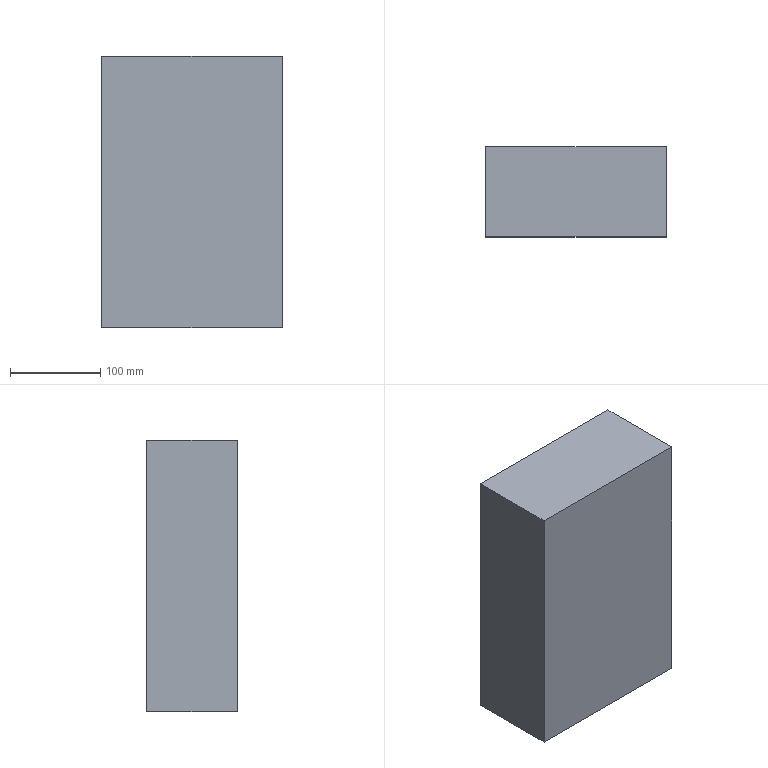Component | SolidWorks | WaterCollectionBox-1 | 1 solid | 11 faces | box 200 x 100 x 300 mm | volume 236864 mm3 | plane 11
build123d program:
from build123d import *

# Parameters (mm, degrees)
SKETCH1_W           = 200
SKETCH1_H           = 300
BOSS_EXTRUDE1_DEPTH = 100
SHELL1_T            = -1.5


with BuildPart() as part:
    # Sketch1 → Boss-Extrude1 (new body)
    with BuildSketch(Plane(origin=(0, 0, 0), x_dir=(1, 0, 0), z_dir=(0, 1, 0))):
        Rectangle(SKETCH1_W, SKETCH1_H)
    extrude(amount=BOSS_EXTRUDE1_DEPTH)

    # Shell1
    shell1_openings = [part.faces().sort_by_distance(p)[0] for p in [
        (0, 100, 0),
    ]]
    offset(amount=SHELL1_T, openings=shell1_openings, kind=Kind.INTERSECTION)


solid = part.part

# Placed as in the assembly
solid = solid.moved(Location((-198.5, 1.5, 0), (0, 0, 0)))
STEP:
#1=CARTESIAN_POINT('',(-3.878,0.05906,5.906));
#2=VERTEX_POINT('',#1);
#3=CARTESIAN_POINT('',(-3.878,0.05906,-5.906));
#4=VERTEX_POINT('',#3);
#5=CARTESIAN_POINT('',(-3.878,0.05906,-5.906));
#6=DIRECTION('',(0.,0.,-1.));
#7=VECTOR('',#6,39.37);
#8=LINE('',#5,#7);
#9=EDGE_CURVE('',#2,#4,#8,.T.);
#10=ORIENTED_EDGE('',*,*,#9,.T.);
#11=CARTESIAN_POINT('',(-3.878,3.996,-5.906));
#12=VERTEX_POINT('',#11);
#13=CARTESIAN_POINT('',(-3.878,3.996,-5.906));
#14=DIRECTION('',(0.,-1.,0.));
#15=VECTOR('',#14,39.37);
#16=LINE('',#13,#15);
#17=EDGE_CURVE('',#12,#4,#16,.T.);
#18=ORIENTED_EDGE('',*,*,#17,.F.);
#19=CARTESIAN_POINT('',(-3.878,3.996,5.906));
#20=VERTEX_POINT('',#19);
#21=CARTESIAN_POINT('',(-3.878,3.996,-5.906));
#22=DIRECTION('',(0.,0.,-1.));
#23=VECTOR('',#22,39.37);
#24=LINE('',#21,#23);
#25=EDGE_CURVE('',#20,#12,#24,.T.);
#26=ORIENTED_EDGE('',*,*,#25,.F.);
#27=CARTESIAN_POINT('',(-3.878,3.996,5.906));
#28=DIRECTION('',(0.,-1.,0.));
#29=VECTOR('',#28,39.37);
#30=LINE('',#27,#29);
#31=EDGE_CURVE('',#20,#2,#30,.T.);
#32=ORIENTED_EDGE('',*,*,#31,.T.);
#33=EDGE_LOOP('',(#10,#18,#26,#32));
#34=FACE_OUTER_BOUND('',#33,.T.);
#35=CARTESIAN_POINT('',(-3.878,3.996,-5.906));
#36=DIRECTION('',(-1.,0.,0.));
#37=DIRECTION('',(0.,0.,1.));
#38=AXIS2_PLACEMENT_3D('',#35,#36,#37);
#39=PLANE('',#38);
#40=ADVANCED_FACE('',(#34),#39,.F.);
#41=CARTESIAN_POINT('',(-11.752,0.05906,-5.906));
#42=VERTEX_POINT('',#41);
#43=CARTESIAN_POINT('',(-11.752,0.05906,-5.906));
#44=DIRECTION('',(-1.,0.,0.));
#45=VECTOR('',#44,39.37);
#46=LINE('',#43,#45);
#47=EDGE_CURVE('',#4,#42,#46,.T.);
#48=ORIENTED_EDGE('',*,*,#47,.T.);
#49=CARTESIAN_POINT('',(-11.752,3.996,-5.906));
#50=VERTEX_POINT('',#49);
#51=CARTESIAN_POINT('',(-11.752,3.996,-5.906));
#52=DIRECTION('',(0.,-1.,0.));
#53=VECTOR('',#52,39.37);
#54=LINE('',#51,#53);
#55=EDGE_CURVE('',#50,#42,#54,.T.);
#56=ORIENTED_EDGE('',*,*,#55,.F.);
#57=CARTESIAN_POINT('',(-11.752,3.996,-5.906));
#58=DIRECTION('',(-1.,0.,0.));
#59=VECTOR('',#58,39.37);
#60=LINE('',#57,#59);
#61=EDGE_CURVE('',#12,#50,#60,.T.);
#62=ORIENTED_EDGE('',*,*,#61,.F.);
#63=ORIENTED_EDGE('',*,*,#17,.T.);
#64=EDGE_LOOP('',(#48,#56,#62,#63));
#65=FACE_OUTER_BOUND('',#64,.T.);
#66=CARTESIAN_POINT('',(-11.752,3.996,-5.906));
#67=DIRECTION('',(0.,0.,1.));
#68=DIRECTION('',(1.,0.,0.));
#69=AXIS2_PLACEMENT_3D('',#66,#67,#68);
#70=PLANE('',#69);
#71=ADVANCED_FACE('',(#65),#70,.F.);
#72=CARTESIAN_POINT('',(-11.752,0.05906,5.906));
#73=VERTEX_POINT('',#72);
#74=CARTESIAN_POINT('',(-11.752,0.05906,-5.906));
#75=DIRECTION('',(0.,0.,1.));
#76=VECTOR('',#75,39.37);
#77=LINE('',#74,#76);
#78=EDGE_CURVE('',#42,#73,#77,.T.);
#79=ORIENTED_EDGE('',*,*,#78,.T.);
#80=CARTESIAN_POINT('',(-11.752,3.996,5.906));
#81=VERTEX_POINT('',#80);
#82=CARTESIAN_POINT('',(-11.752,3.996,5.906));
#83=DIRECTION('',(0.,-1.,0.));
#84=VECTOR('',#83,39.37);
#85=LINE('',#82,#84);
#86=EDGE_CURVE('',#81,#73,#85,.T.);
#87=ORIENTED_EDGE('',*,*,#86,.F.);
#88=CARTESIAN_POINT('',(-11.752,3.996,-5.906));
#89=DIRECTION('',(0.,0.,1.));
#90=VECTOR('',#89,39.37);
#91=LINE('',#88,#90);
#92=EDGE_CURVE('',#50,#81,#91,.T.);
#93=ORIENTED_EDGE('',*,*,#92,.F.);
#94=ORIENTED_EDGE('',*,*,#55,.T.);
#95=EDGE_LOOP('',(#79,#87,#93,#94));
#96=FACE_OUTER_BOUND('',#95,.T.);
#97=CARTESIAN_POINT('',(-11.752,3.996,-5.906));
#98=DIRECTION('',(1.,0.,0.));
#99=DIRECTION('',(0.,0.,-1.));
#100=AXIS2_PLACEMENT_3D('',#97,#98,#99);
#101=PLANE('',#100);
#102=ADVANCED_FACE('',(#96),#101,.F.);
#103=CARTESIAN_POINT('',(-11.752,0.05906,5.906));
#104=DIRECTION('',(1.,0.,0.));
#105=VECTOR('',#104,39.37);
#106=LINE('',#103,#105);
#107=EDGE_CURVE('',#73,#2,#106,.T.);
#108=ORIENTED_EDGE('',*,*,#107,.T.);
#109=ORIENTED_EDGE('',*,*,#31,.F.);
#110=CARTESIAN_POINT('',(-11.752,3.996,5.906));
#111=DIRECTION('',(1.,0.,0.));
#112=VECTOR('',#111,39.37);
#113=LINE('',#110,#112);
#114=EDGE_CURVE('',#81,#20,#113,.T.);
#115=ORIENTED_EDGE('',*,*,#114,.F.);
#116=ORIENTED_EDGE('',*,*,#86,.T.);
#117=EDGE_LOOP('',(#108,#109,#115,#116));
#118=FACE_OUTER_BOUND('',#117,.T.);
#119=CARTESIAN_POINT('',(-11.752,3.996,5.906));
#120=DIRECTION('',(0.,0.,-1.));
#121=DIRECTION('',(-1.,0.,0.));
#122=AXIS2_PLACEMENT_3D('',#119,#120,#121);
#123=PLANE('',#122);
#124=ADVANCED_FACE('',(#118),#123,.F.);
#125=CARTESIAN_POINT('',(-3.937,3.996,5.846));
#126=VERTEX_POINT('',#125);
#127=CARTESIAN_POINT('',(-3.937,3.996,-5.846));
#128=VERTEX_POINT('',#127);
#129=CARTESIAN_POINT('',(-3.937,3.996,-5.906));
#130=DIRECTION('',(0.,0.,-1.));
#131=VECTOR('',#130,39.37);
#132=LINE('',#129,#131);
#133=EDGE_CURVE('',#126,#128,#132,.T.);
#134=ORIENTED_EDGE('',*,*,#133,.F.);
#135=CARTESIAN_POINT('',(-11.693,3.996,5.846));
#136=VERTEX_POINT('',#135);
#137=CARTESIAN_POINT('',(-11.752,3.996,5.846));
#138=DIRECTION('',(1.,0.,0.));
#139=VECTOR('',#138,39.37);
#140=LINE('',#137,#139);
#141=EDGE_CURVE('',#136,#126,#140,.T.);
#142=ORIENTED_EDGE('',*,*,#141,.F.);
#143=CARTESIAN_POINT('',(-11.693,3.996,-5.846));
#144=VERTEX_POINT('',#143);
#145=CARTESIAN_POINT('',(-11.693,3.996,-5.906));
#146=DIRECTION('',(0.,0.,1.));
#147=VECTOR('',#146,39.37);
#148=LINE('',#145,#147);
#149=EDGE_CURVE('',#144,#136,#148,.T.);
#150=ORIENTED_EDGE('',*,*,#149,.F.);
#151=CARTESIAN_POINT('',(-11.752,3.996,-5.846));
#152=DIRECTION('',(-1.,0.,0.));
#153=VECTOR('',#152,39.37);
#154=LINE('',#151,#153);
#155=EDGE_CURVE('',#128,#144,#154,.T.);
#156=ORIENTED_EDGE('',*,*,#155,.F.);
#157=EDGE_LOOP('',(#134,#142,#150,#156));
#158=FACE_BOUND('',#157,.T.);
#159=ORIENTED_EDGE('',*,*,#25,.T.);
#160=ORIENTED_EDGE('',*,*,#61,.T.);
#161=ORIENTED_EDGE('',*,*,#92,.T.);
#162=ORIENTED_EDGE('',*,*,#114,.T.);
#163=EDGE_LOOP('',(#159,#160,#161,#162));
#164=FACE_OUTER_BOUND('',#163,.T.);
#165=CARTESIAN_POINT('',(-7.815,3.996,-0.));
#166=DIRECTION('',(0.,1.,0.));
#167=DIRECTION('',(0.,0.,1.));
#168=AXIS2_PLACEMENT_3D('',#165,#166,#167);
#169=PLANE('',#168);
#170=ADVANCED_FACE('',(#158,#164),#169,.T.);
#171=ORIENTED_EDGE('',*,*,#9,.F.);
#172=ORIENTED_EDGE('',*,*,#107,.F.);
#173=ORIENTED_EDGE('',*,*,#78,.F.);
#174=ORIENTED_EDGE('',*,*,#47,.F.);
#175=EDGE_LOOP('',(#171,#172,#173,#174));
#176=FACE_OUTER_BOUND('',#175,.T.);
#177=CARTESIAN_POINT('',(-7.815,0.05906,-0.));
#178=DIRECTION('',(0.,1.,0.));
#179=DIRECTION('',(0.,0.,1.));
#180=AXIS2_PLACEMENT_3D('',#177,#178,#179);
#181=PLANE('',#180);
#182=ADVANCED_FACE('',(#176),#181,.F.);
#183=CARTESIAN_POINT('',(-3.937,0.1181,5.846));
#184=VERTEX_POINT('',#183);
#185=CARTESIAN_POINT('',(-3.937,0.1181,-5.846));
#186=VERTEX_POINT('',#185);
#187=CARTESIAN_POINT('',(-3.937,0.1181,-5.906));
#188=DIRECTION('',(0.,0.,-1.));
#189=VECTOR('',#188,39.37);
#190=LINE('',#187,#189);
#191=EDGE_CURVE('',#184,#186,#190,.T.);
#192=ORIENTED_EDGE('',*,*,#191,.F.);
#193=CARTESIAN_POINT('',(-3.937,3.996,5.846));
#194=DIRECTION('',(0.,-1.,0.));
#195=VECTOR('',#194,39.37);
#196=LINE('',#193,#195);
#197=EDGE_CURVE('',#126,#184,#196,.T.);
#198=ORIENTED_EDGE('',*,*,#197,.F.);
#199=ORIENTED_EDGE('',*,*,#133,.T.);
#200=CARTESIAN_POINT('',(-3.937,3.996,-5.846));
#201=DIRECTION('',(0.,-1.,0.));
#202=VECTOR('',#201,39.37);
#203=LINE('',#200,#202);
#204=EDGE_CURVE('',#128,#186,#203,.T.);
#205=ORIENTED_EDGE('',*,*,#204,.T.);
#206=EDGE_LOOP('',(#192,#198,#199,#205));
#207=FACE_OUTER_BOUND('',#206,.T.);
#208=CARTESIAN_POINT('',(-3.937,3.996,-5.906));
#209=DIRECTION('',(-1.,0.,0.));
#210=DIRECTION('',(0.,0.,1.));
#211=AXIS2_PLACEMENT_3D('',#208,#209,#210);
#212=PLANE('',#211);
#213=ADVANCED_FACE('',(#207),#212,.T.);
#214=CARTESIAN_POINT('',(-11.693,0.1181,-5.846));
#215=VERTEX_POINT('',#214);
#216=CARTESIAN_POINT('',(-11.752,0.1181,-5.846));
#217=DIRECTION('',(-1.,0.,0.));
#218=VECTOR('',#217,39.37);
#219=LINE('',#216,#218);
#220=EDGE_CURVE('',#186,#215,#219,.T.);
#221=ORIENTED_EDGE('',*,*,#220,.F.);
#222=ORIENTED_EDGE('',*,*,#204,.F.);
#223=ORIENTED_EDGE('',*,*,#155,.T.);
#224=CARTESIAN_POINT('',(-11.693,3.996,-5.846));
#225=DIRECTION('',(0.,-1.,0.));
#226=VECTOR('',#225,39.37);
#227=LINE('',#224,#226);
#228=EDGE_CURVE('',#144,#215,#227,.T.);
#229=ORIENTED_EDGE('',*,*,#228,.T.);
#230=EDGE_LOOP('',(#221,#222,#223,#229));
#231=FACE_OUTER_BOUND('',#230,.T.);
#232=CARTESIAN_POINT('',(-11.752,3.996,-5.846));
#233=DIRECTION('',(0.,0.,1.));
#234=DIRECTION('',(1.,0.,0.));
#235=AXIS2_PLACEMENT_3D('',#232,#233,#234);
#236=PLANE('',#235);
#237=ADVANCED_FACE('',(#231),#236,.T.);
#238=CARTESIAN_POINT('',(-11.693,0.1181,5.846));
#239=VERTEX_POINT('',#238);
#240=CARTESIAN_POINT('',(-11.693,0.1181,-5.906));
#241=DIRECTION('',(0.,0.,1.));
#242=VECTOR('',#241,39.37);
#243=LINE('',#240,#242);
#244=EDGE_CURVE('',#215,#239,#243,.T.);
#245=ORIENTED_EDGE('',*,*,#244,.F.);
#246=ORIENTED_EDGE('',*,*,#228,.F.);
#247=ORIENTED_EDGE('',*,*,#149,.T.);
#248=CARTESIAN_POINT('',(-11.693,3.996,5.846));
#249=DIRECTION('',(0.,-1.,0.));
#250=VECTOR('',#249,39.37);
#251=LINE('',#248,#250);
#252=EDGE_CURVE('',#136,#239,#251,.T.);
#253=ORIENTED_EDGE('',*,*,#252,.T.);
#254=EDGE_LOOP('',(#245,#246,#247,#253));
#255=FACE_OUTER_BOUND('',#254,.T.);
#256=CARTESIAN_POINT('',(-11.693,3.996,-5.906));
#257=DIRECTION('',(1.,0.,0.));
#258=DIRECTION('',(0.,0.,-1.));
#259=AXIS2_PLACEMENT_3D('',#256,#257,#258);
#260=PLANE('',#259);
#261=ADVANCED_FACE('',(#255),#260,.T.);
#262=CARTESIAN_POINT('',(-11.752,0.1181,5.846));
#263=DIRECTION('',(1.,0.,0.));
#264=VECTOR('',#263,39.37);
#265=LINE('',#262,#264);
#266=EDGE_CURVE('',#239,#184,#265,.T.);
#267=ORIENTED_EDGE('',*,*,#266,.F.);
#268=ORIENTED_EDGE('',*,*,#252,.F.);
#269=ORIENTED_EDGE('',*,*,#141,.T.);
#270=ORIENTED_EDGE('',*,*,#197,.T.);
#271=EDGE_LOOP('',(#267,#268,#269,#270));
#272=FACE_OUTER_BOUND('',#271,.T.);
#273=CARTESIAN_POINT('',(-11.752,3.996,5.846));
#274=DIRECTION('',(0.,0.,-1.));
#275=DIRECTION('',(-1.,0.,0.));
#276=AXIS2_PLACEMENT_3D('',#273,#274,#275);
#277=PLANE('',#276);
#278=ADVANCED_FACE('',(#272),#277,.T.);
#279=ORIENTED_EDGE('',*,*,#191,.T.);
#280=ORIENTED_EDGE('',*,*,#220,.T.);
#281=ORIENTED_EDGE('',*,*,#244,.T.);
#282=ORIENTED_EDGE('',*,*,#266,.T.);
#283=EDGE_LOOP('',(#279,#280,#281,#282));
#284=FACE_OUTER_BOUND('',#283,.T.);
#285=CARTESIAN_POINT('',(-7.815,0.1181,-0.));
#286=DIRECTION('',(0.,1.,0.));
#287=DIRECTION('',(0.,0.,1.));
#288=AXIS2_PLACEMENT_3D('',#285,#286,#287);
#289=PLANE('',#288);
#290=ADVANCED_FACE('',(#284),#289,.T.);
#291=CLOSED_SHELL('',(#40,#71,#102,#124,#170,#182,#213,#237,#261,#278,#290));
#292=MANIFOLD_SOLID_BREP('',#291);
#293=CARTESIAN_POINT('',(0.,0.,0.));
#294=DIRECTION('',(0.,0.,1.));
#295=DIRECTION('',(1.,0.,0.));
#296=AXIS2_PLACEMENT_3D('',#293,#294,#295);
#297=(LENGTH_UNIT()NAMED_UNIT(*)SI_UNIT($,.METRE.));
#298=LENGTH_MEASURE_WITH_UNIT(LENGTH_MEASURE(0.0254),#297);
#299=DIMENSIONAL_EXPONENTS(1.,0.,0.,0.,0.,0.,0.);
#300=(CONVERSION_BASED_UNIT('',#298)LENGTH_UNIT()NAMED_UNIT(#299));
#301=UNCERTAINTY_MEASURE_WITH_UNIT(LENGTH_MEASURE(0.00001),#300,'','');
#302=(NAMED_UNIT(*)PLANE_ANGLE_UNIT()SI_UNIT($,.RADIAN.));
#303=(NAMED_UNIT(*)SI_UNIT($,.STERADIAN.)SOLID_ANGLE_UNIT());
#304=(GEOMETRIC_REPRESENTATION_CONTEXT(3)GLOBAL_UNCERTAINTY_ASSIGNED_CONTEXT((#301))GLOBAL_UNIT_ASSIGNED_CONTEXT((#300,#302,#303))REPRESENTATION_CONTEXT('',''));
#305=ADVANCED_BREP_SHAPE_REPRESENTATION('',(#292,#296),#304);
#306=COLOUR_RGB('',0.7922,0.8196,0.9333);
#307=FILL_AREA_STYLE_COLOUR('',#306);
#308=FILL_AREA_STYLE('',(#307));
#309=SURFACE_STYLE_FILL_AREA(#308);
#310=SURFACE_SIDE_STYLE('',(#309));
#311=SURFACE_STYLE_USAGE(.BOTH.,#310);
#312=PRESENTATION_STYLE_ASSIGNMENT((#311));
#313=STYLED_ITEM('',(#312),#292);
#314=PRESENTATION_LAYER_ASSIGNMENT('','',(#313));
#315=(LENGTH_UNIT()NAMED_UNIT(*)SI_UNIT($,.METRE.));
#316=LENGTH_MEASURE_WITH_UNIT(LENGTH_MEASURE(0.0254),#315);
#317=DIMENSIONAL_EXPONENTS(1.,0.,0.,0.,0.,0.,0.);
#318=(CONVERSION_BASED_UNIT('',#316)LENGTH_UNIT()NAMED_UNIT(#317));
#319=UNCERTAINTY_MEASURE_WITH_UNIT(LENGTH_MEASURE(0.00001),#318,'','');
#320=(NAMED_UNIT(*)PLANE_ANGLE_UNIT()SI_UNIT($,.RADIAN.));
#321=(NAMED_UNIT(*)SI_UNIT($,.STERADIAN.)SOLID_ANGLE_UNIT());
#322=(GEOMETRIC_REPRESENTATION_CONTEXT(3)GLOBAL_UNCERTAINTY_ASSIGNED_CONTEXT((#319))GLOBAL_UNIT_ASSIGNED_CONTEXT((#318,#320,#321))REPRESENTATION_CONTEXT('',''));
#323=MECHANICAL_DESIGN_GEOMETRIC_PRESENTATION_REPRESENTATION('',(#313),#322);